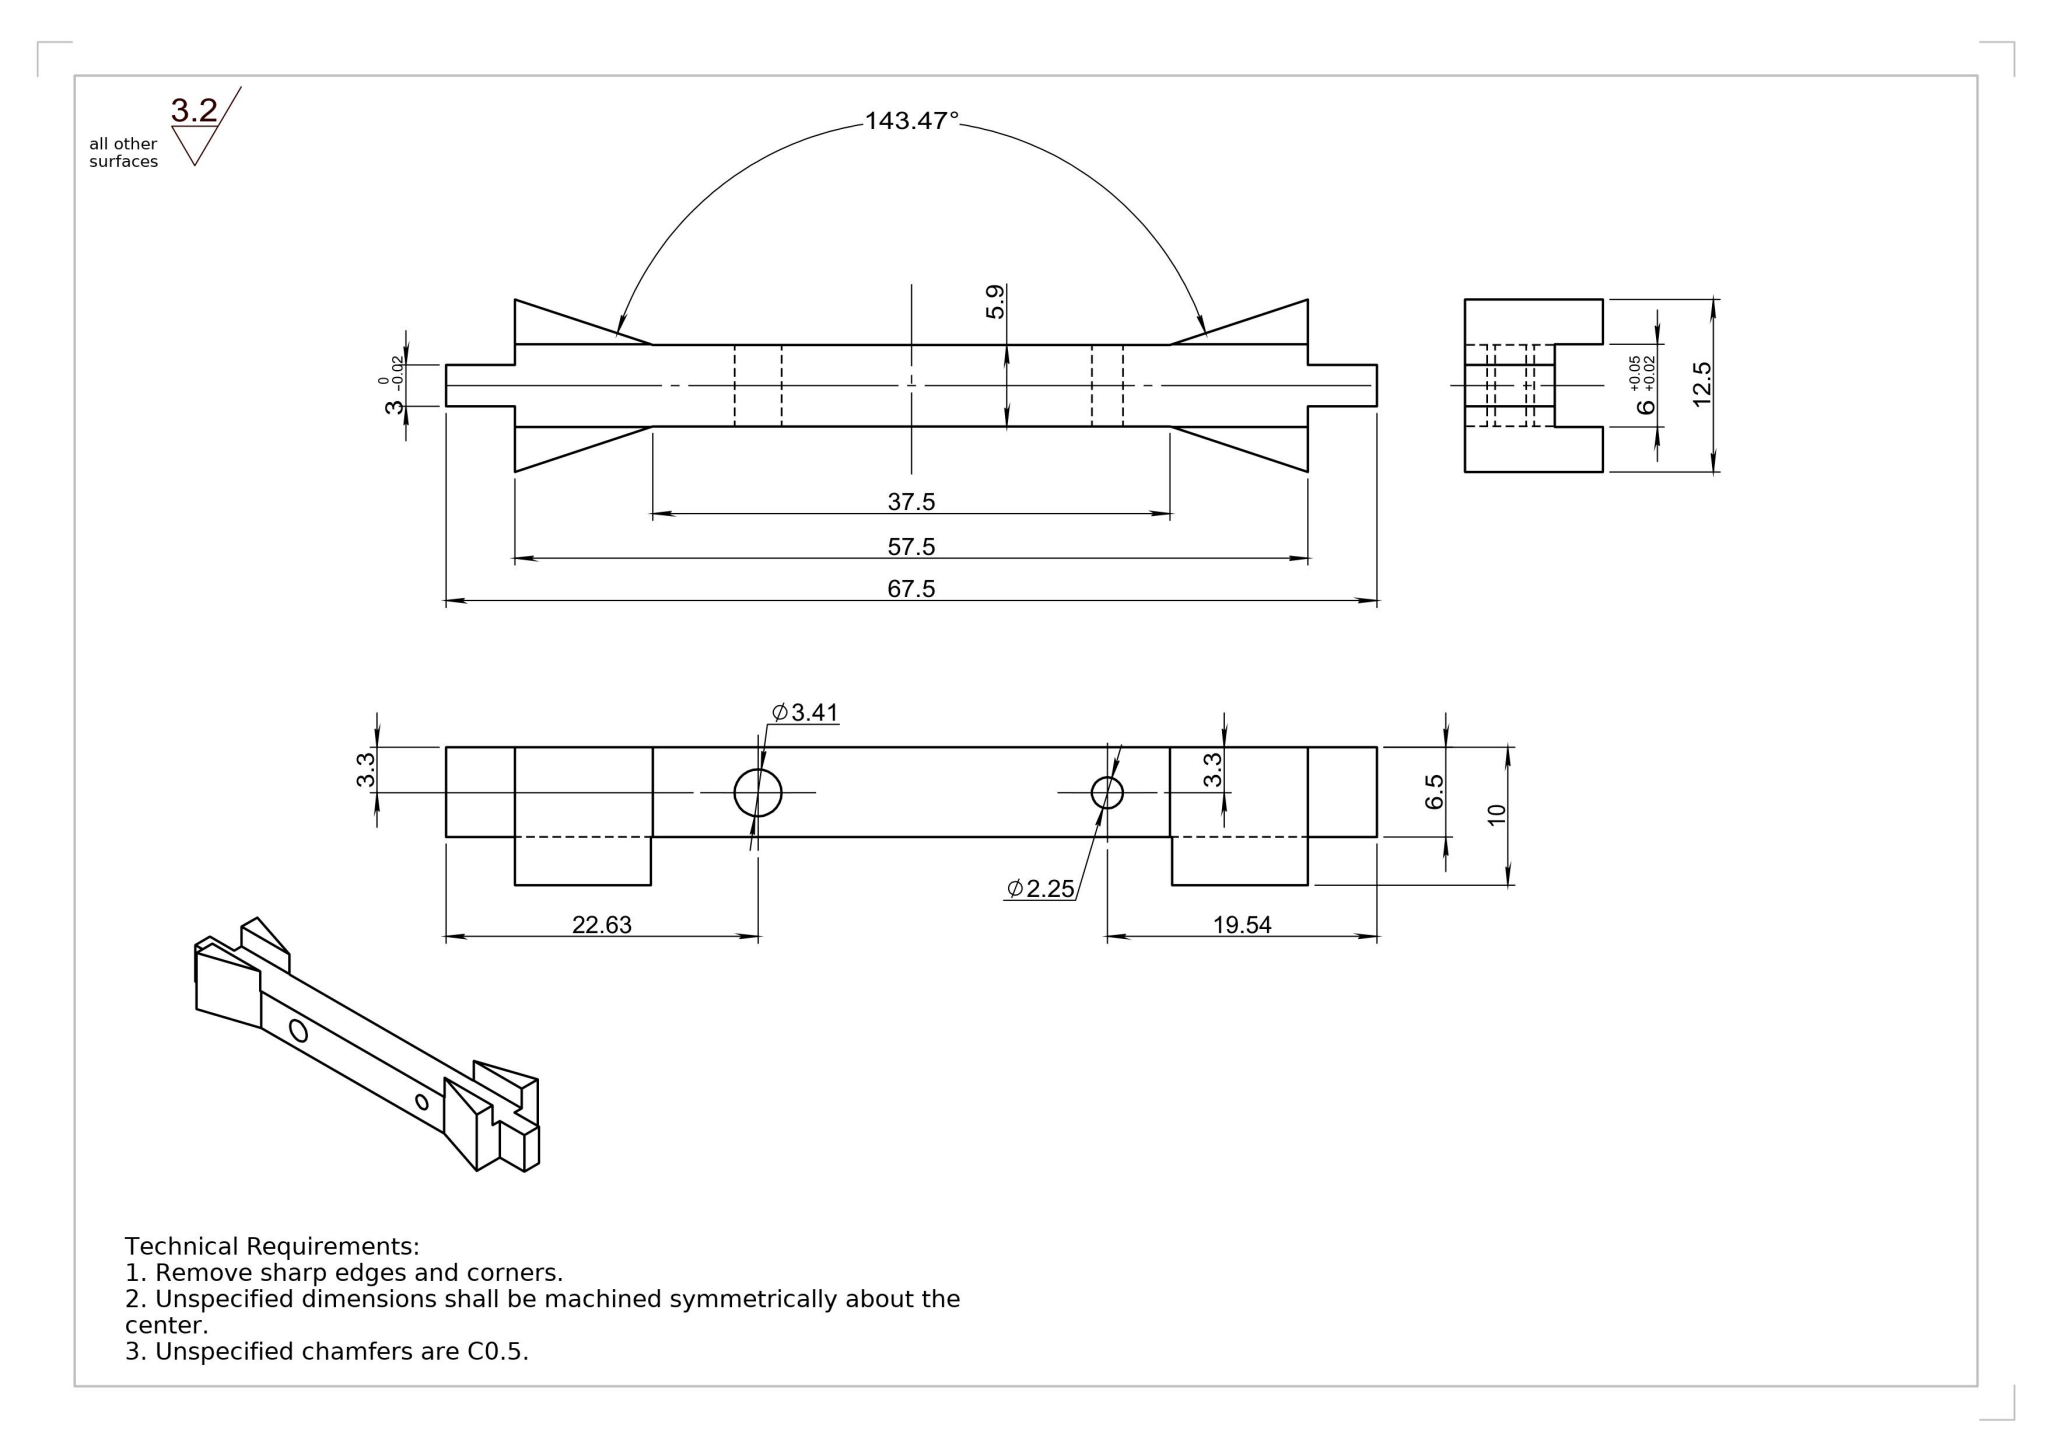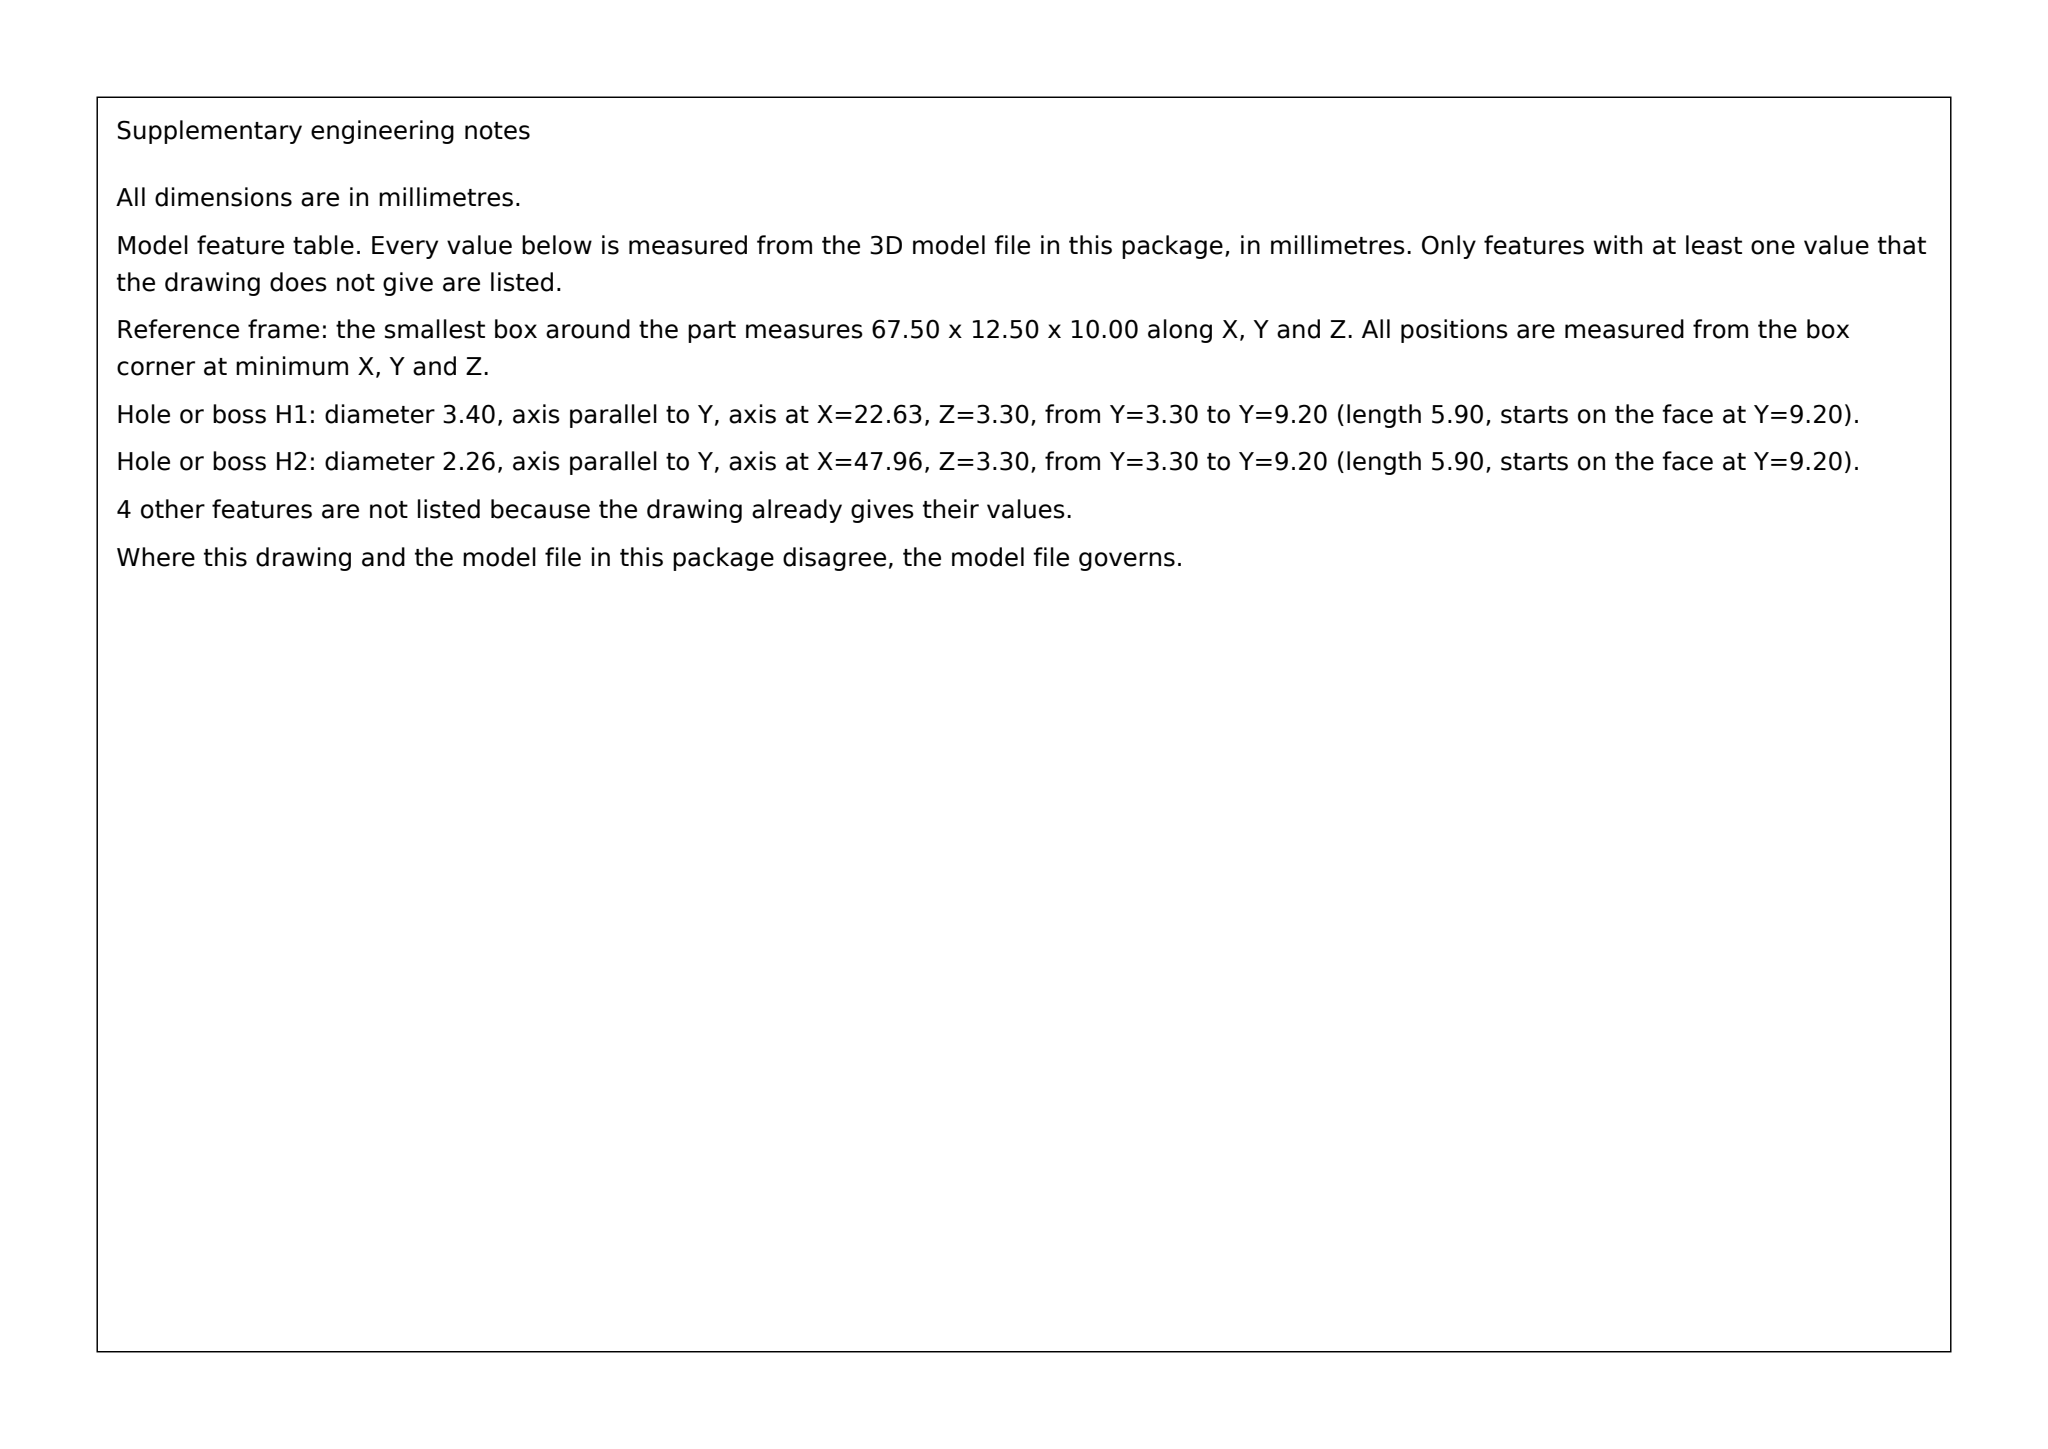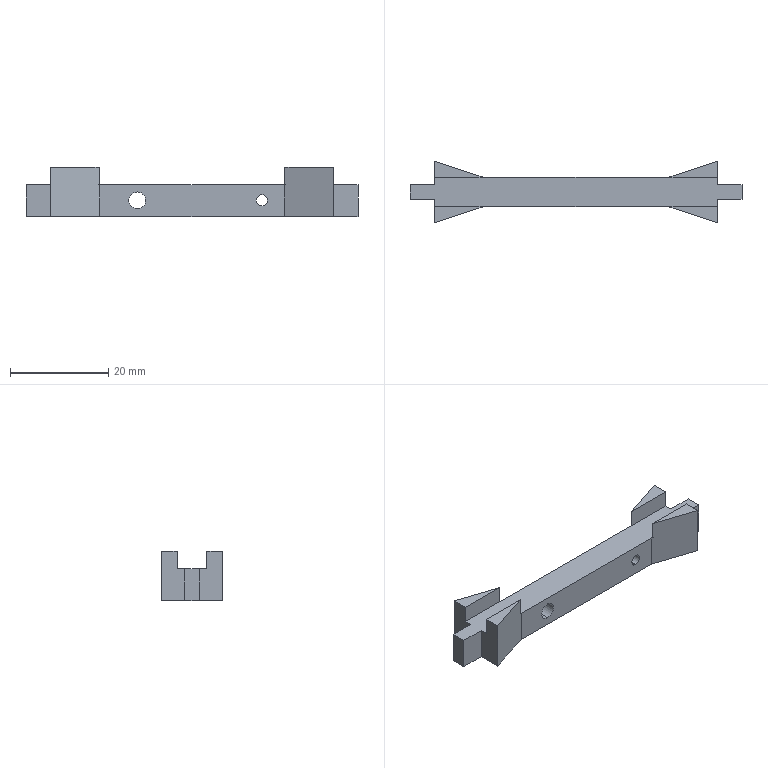Part | SolidWorks | mm | 1 solid | 30 faces | box 67.5 x 12.5 x 10 mm | volume 2976 mm3 | plane 26 | cylinder 4 | commonest cylinder face diameters 3.408 x2 2.255 x2
build123d program:
from build123d import *

# Parameters (mm, degrees)
BOSS_EXTRUDE1_DEPTH = 10
SKETCH2_W           = 73.258
SKETCH2_H           = 6
CUT_EXTRUDE1_DEPTH  = 3.5
SKETCH3_R           = 1.704
SKETCH3_R_2         = 1.127
CUT_EXTRUDE2_DEPTH  = 80


with BuildPart() as part:
    # Sketch1 → Boss-Extrude1 (new body)
    with BuildSketch(Plane.XY):
        Polygon((-18.75, 2.95), (-28.75, 6.25), (-28.75, 1.5), (-33.75, 1.5), (-33.75, -1.5), (-28.75, -1.5), (-28.75, -6.25), (-18.75, -2.95), (18.75, -2.95), (28.75, -6.25), (28.75, -1.5), (33.75, -1.5), (33.75, 1.5), (28.75, 1.5), (28.75, 6.25), (18.75, 2.95), align=None)
    extrude(amount=BOSS_EXTRUDE1_DEPTH)

    # Sketch2 → Cut-Extrude1 (cut)
    with BuildSketch(Plane.XY.offset(10)):
        Rectangle(SKETCH2_W, SKETCH2_H)
    extrude(amount=-CUT_EXTRUDE1_DEPTH, mode=Mode.SUBTRACT)

    # Sketch3 → Cut-Extrude2 (cut)
    with BuildSketch(Plane(origin=(0, 2.95, 0), x_dir=(1, 0, 0), z_dir=(0, 1, 0))):
        with Locations(Location((-11.125, -3.299, 0), (0, 0, 270))):
            Circle(SKETCH3_R)
        with Locations(Location((14.206, -3.299, 0), (0, 0, 270))):
            Circle(SKETCH3_R_2)
    extrude(amount=-CUT_EXTRUDE2_DEPTH, mode=Mode.SUBTRACT)


solid = part.part